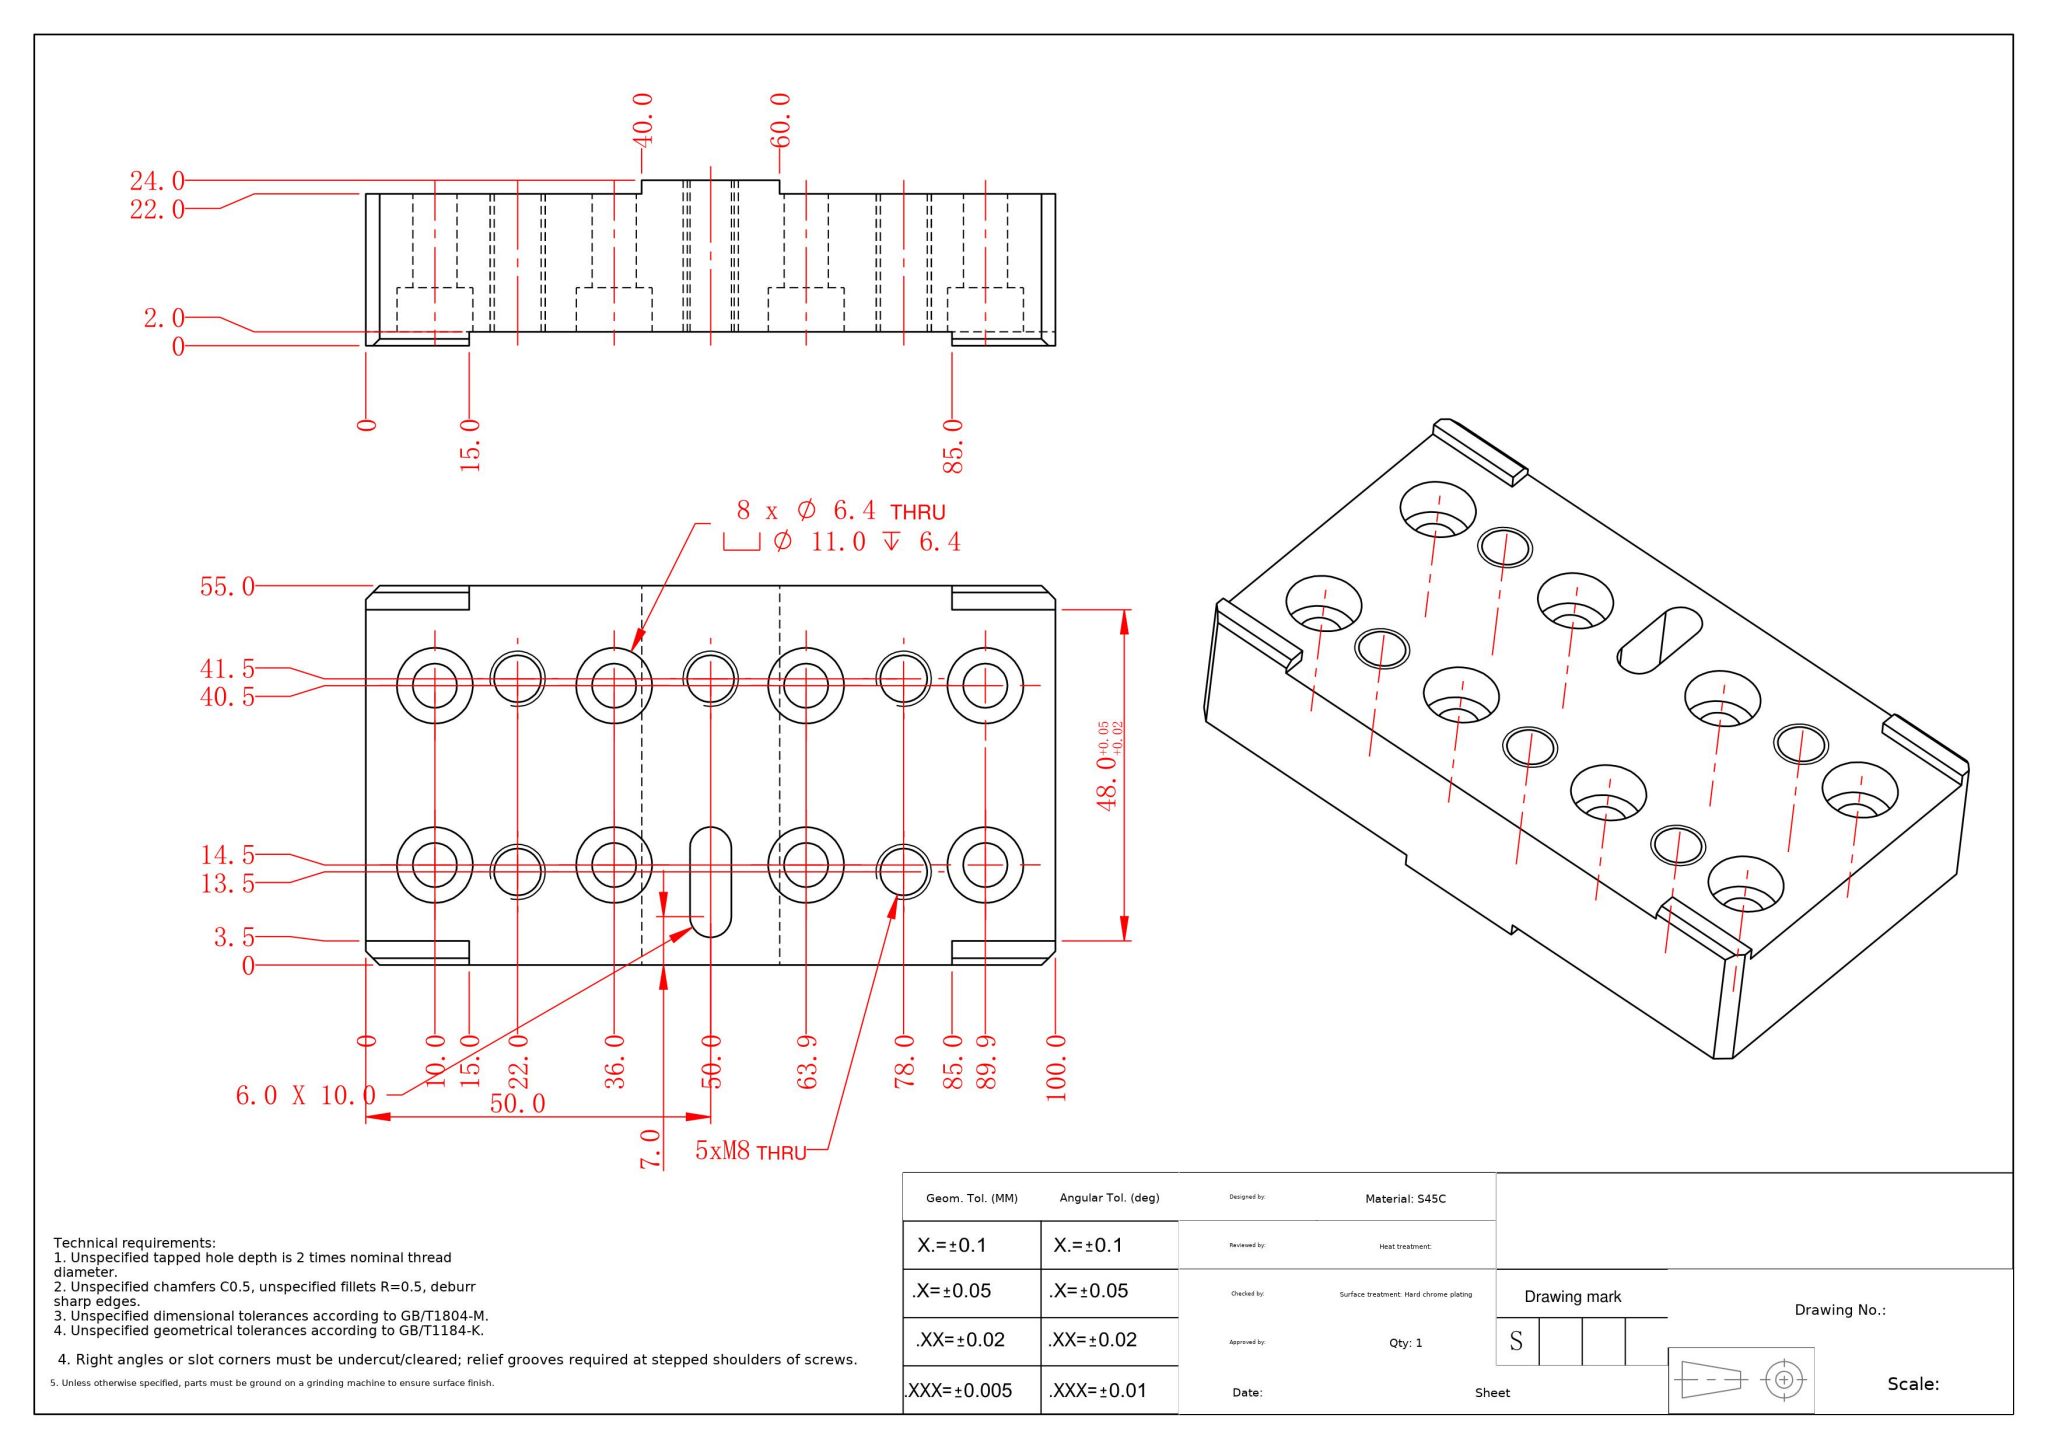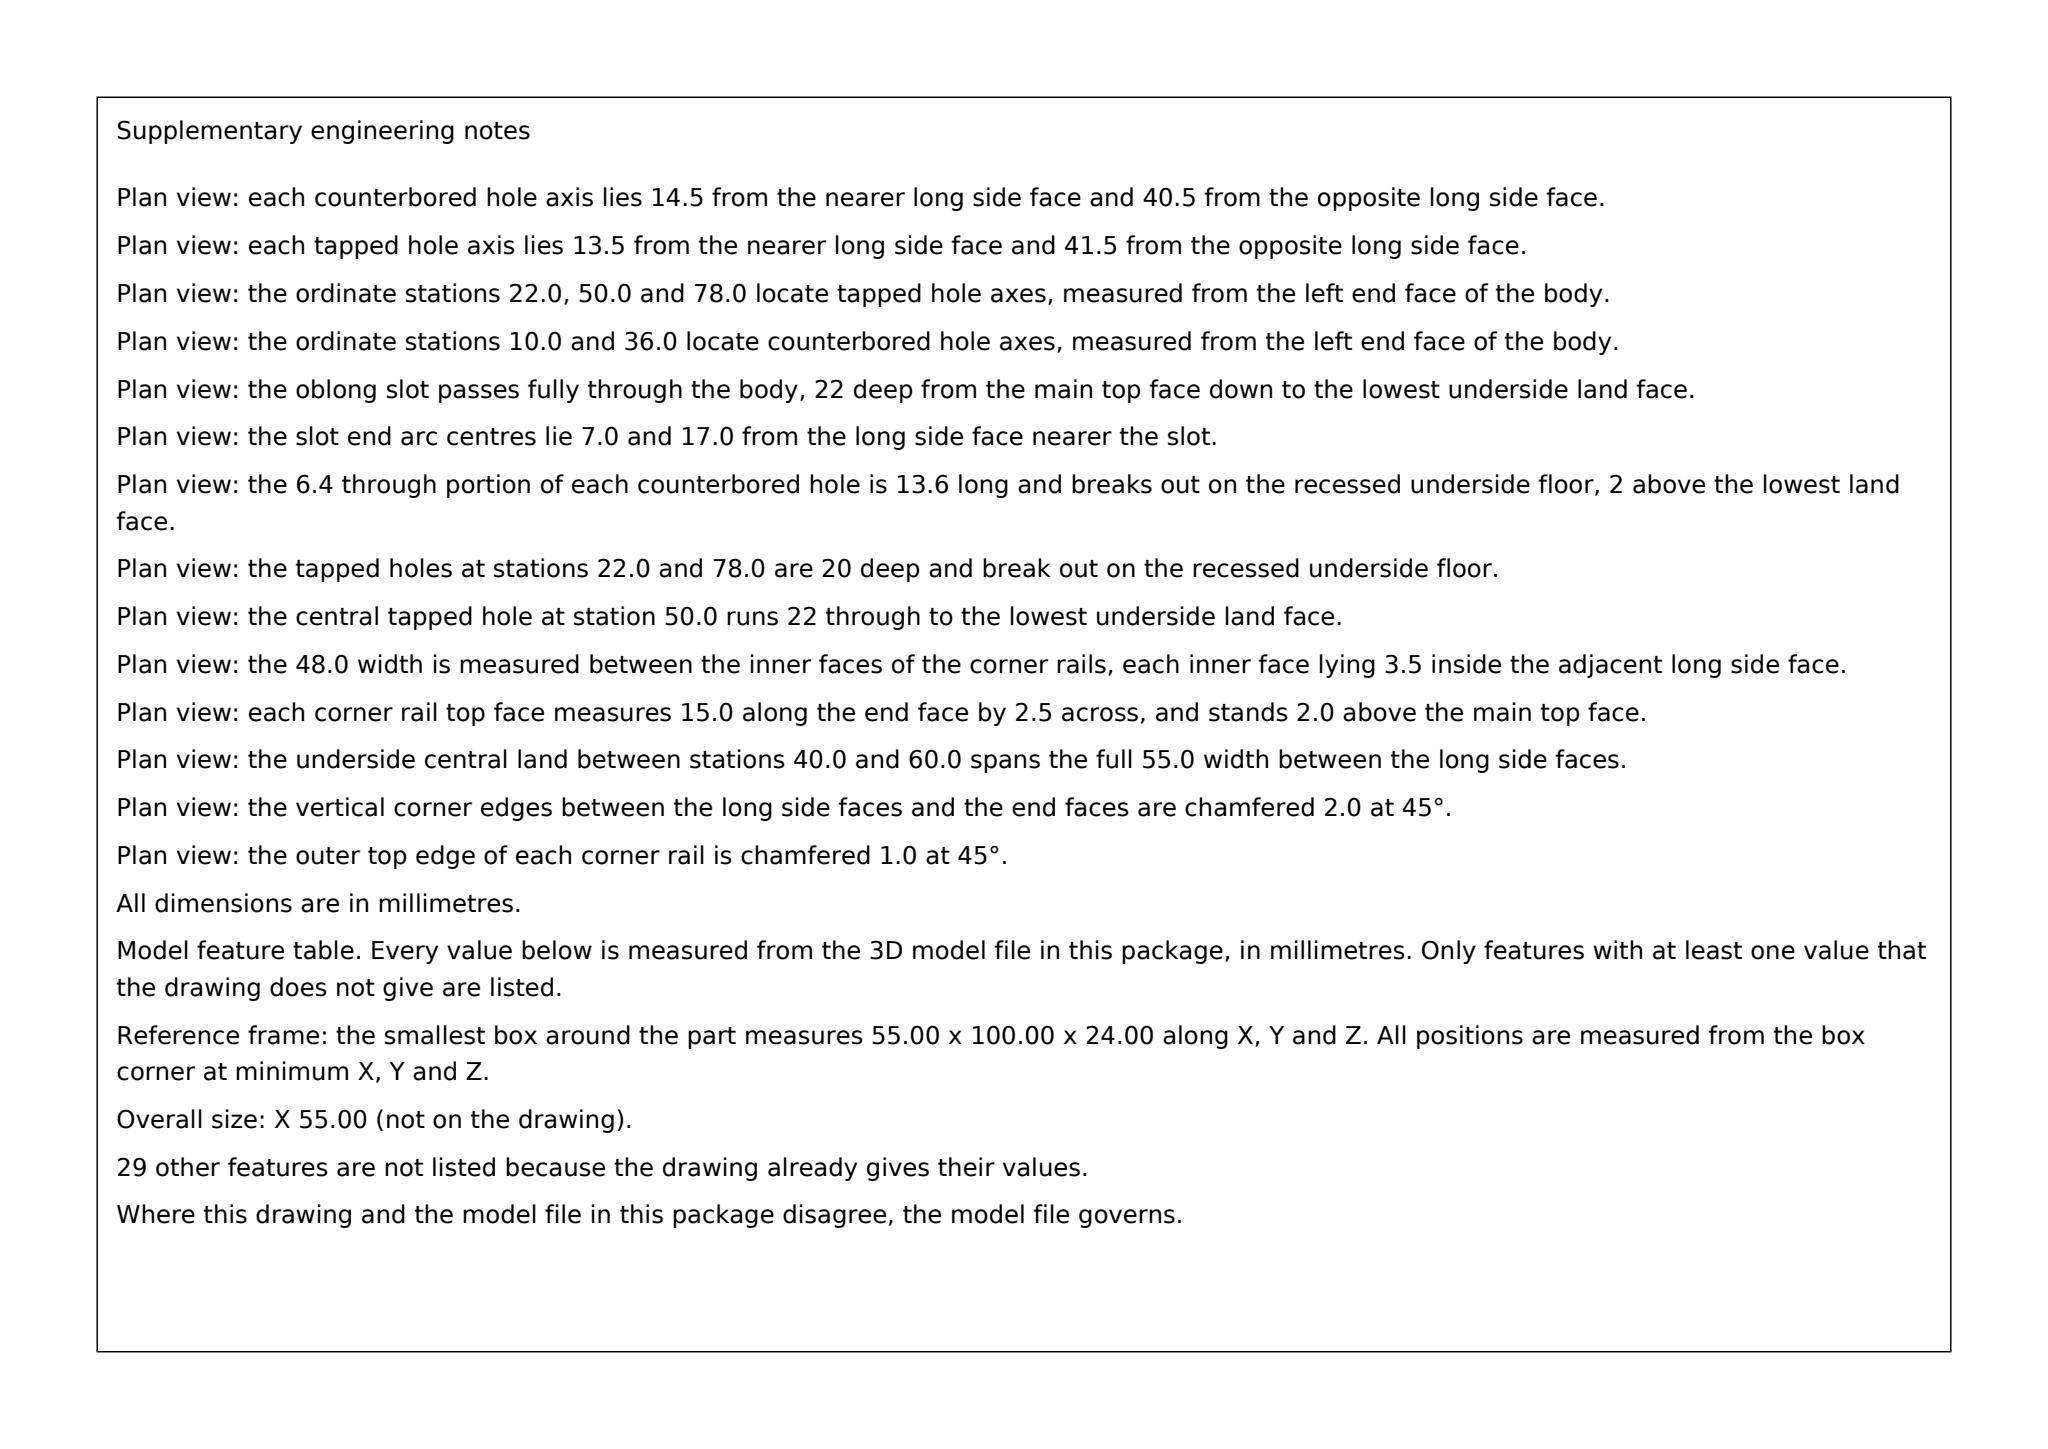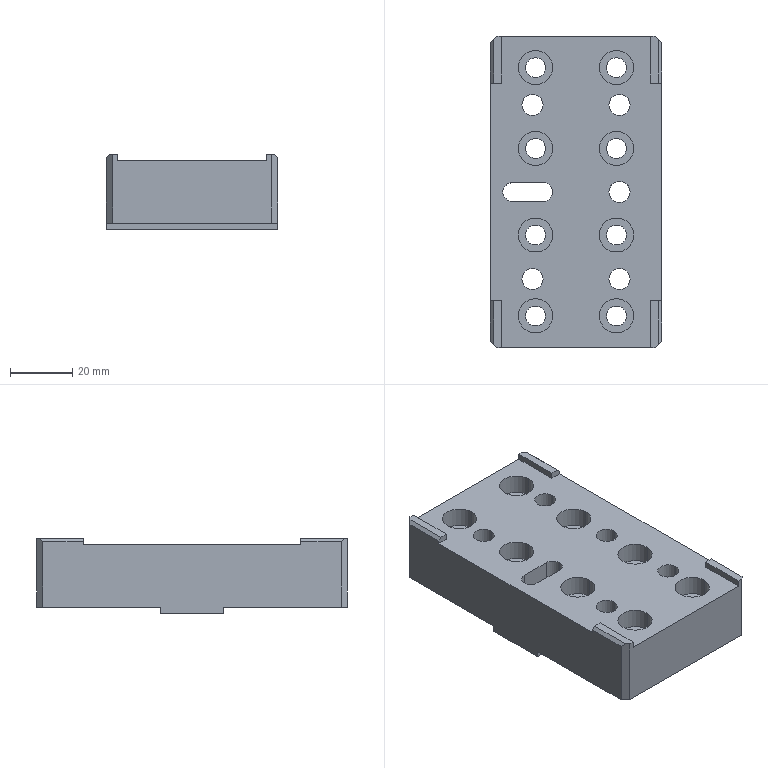Part | SolidWorks | mm | 1 solid | 85 faces | box 55 x 100 x 24 mm | volume 98405 mm3 | cylinder 45 | plane 40 | commonest cylinder face diameters 11 x16 6.4 x16 6.8 x10 6 x3
Drawing notes:
8X Ø6.4 THRU CBORE ON CL 14.5 & 40.5 FROM BTM EDGE | from the solid: Ø6.4/Ø11.0 cyls at x=14.5 and x=40.5 (bbox min corner datum)
5X M8 THRU ON CL 13.5 & 41.5 FROM BTM EDGE | from the solid: Ø6.8 tap drill cyls at x=13.5 and x=41.5
ROW SPACING 26.0 (14.5 TO 40.5) & 28.0 (13.5 TO 41.5) | from the solid: x-positions 14.5/40.5 and 13.5/41.5
6.0 X 10.0 SLOT THRU 22.0, CL 12.0 FROM BTM EDGE AT Y50.0 | from the solid: Two Ø6.0 z-cyls at (7.0,50.0) & (17.0,50.0), length 22.0 = full 22.0 thk (z 0-22)
8X Ø6.4 THRU, CBORE Ø11.0 DP 6.4 FROM TOP FACE (Z=22.0) | from the solid: Counterbore openings appear on upper face in isometric; top face at 22.0 above Z0 datum (front view), bore depth 6.4 measured down from it